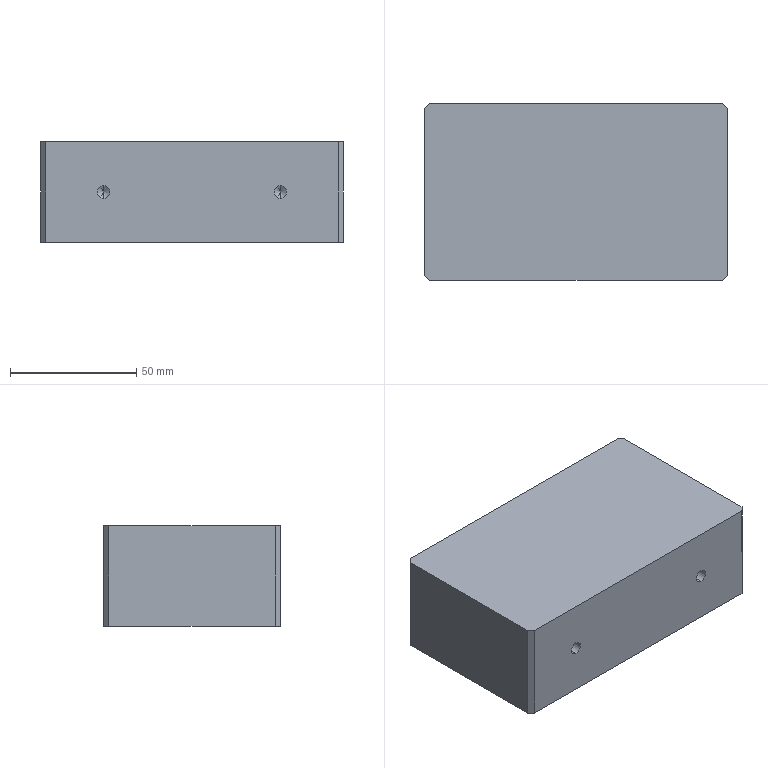Component | SolidWorks | ThirdGenerationFour-sidedLabelingFeedingSupportPlate-1 | 1 solid | 34 faces | box 120 x 70 x 40 mm | volume 334028 mm3 | cylinder 12 | cone 12 | plane 10 | commonest cylinder face diameters 4.2 x8 5 x4
build123d program:
from build123d import *

# Parameters (mm, degrees)
SKETCH1_W                  = 120
SKETCH1_H                  = 70
BOSS_EXTRUDE1_DEPTH        = 20
M5_TAPPED_HOLE1_AT_2_COUNT = 2
M5_TAPPED_HOLE1_AT_2_PITCH = 100
M6_TAPPED_HOLE1_AT_2_COUNT = 2
M6_TAPPED_HOLE1_AT_2_PITCH = 70
CHAMFER1_SIZE              = 2


with BuildPart() as part:
    # Sketch1 → Boss-Extrude1 (new, symmetric)
    with BuildSketch(Plane.XY):
        Rectangle(SKETCH1_W, SKETCH1_H)
    extrude(amount=BOSS_EXTRUDE1_DEPTH, both=True)

    # Sketch2 → M5 Tapped Hole1 (revolve, cut)
    with BuildSketch(Plane(origin=(-50, 35, -12), x_dir=(0, 0, 1), z_dir=(1, 0, 0))):
        Polygon((0, 0), (0, 19.662), (2.1, 18.4), (2.1, 0), align=None)
    m5_tapped_hole1 = revolve(axis=Axis((-50, 41.35, -12), (0, -1, 0)), mode=Mode.SUBTRACT)

    # M5 Tapped Hole1 at 2: M5 Tapped Hole1 ×2
    with Locations(*[(i * M5_TAPPED_HOLE1_AT_2_PITCH, 0, 0) for i in range(1, M5_TAPPED_HOLE1_AT_2_COUNT)]):
        add(m5_tapped_hole1, mode=Mode.SUBTRACT)

    # Sketch5 → M6 Tapped Hole1 (revolve, cut)
    with BuildSketch(Plane(origin=(-35, -35, 0), x_dir=(0, 0, -1), z_dir=(1, 0, 0))):
        Polygon((0, 0), (0, 16.502), (2.5, 15), (2.5, 0), align=None)
    m6_tapped_hole1 = revolve(axis=Axis((-35, -41.35, 0), (0, 1, 0)), mode=Mode.SUBTRACT)

    # M6 Tapped Hole1 at 2: M6 Tapped Hole1 ×2
    with Locations(*[(i * M6_TAPPED_HOLE1_AT_2_PITCH, 0, 0) for i in range(1, M6_TAPPED_HOLE1_AT_2_COUNT)]):
        add(m6_tapped_hole1, mode=Mode.SUBTRACT)

    # Chamfer1
    chamfer1_edges = [part.edges().sort_by_distance(p)[0] for p in [
        (60, -35, 0),
        (-60, -35, 0),
        (-60, 35, 0),
        (60, 35, 0),
    ]]
    chamfer(chamfer1_edges, length=CHAMFER1_SIZE)

    # Mirror1: M5 Tapped Hole1, M6 Tapped Hole1 across plane
    add(m5_tapped_hole1.mirror(Plane.XY), mode=Mode.SUBTRACT)
    add(m6_tapped_hole1.mirror(Plane.XY), mode=Mode.SUBTRACT)

    # Mirror1 copy 1 sketch → Mirror1 copy 1 (revolve, cut)
    with BuildSketch(Plane(origin=(50, 35, 12), x_dir=(0, 0, -1), z_dir=(1, 0, 0))):
        Polygon((0, 0), (0, -19.662), (2.1, -18.4), (2.1, 0), align=None)
    revolve(axis=Axis((50, 41.35, 12), (0, 1, 0)), mode=Mode.SUBTRACT)

    # Mirror1 copy 2 sketch → Mirror1 copy 2 (revolve, cut)
    with BuildSketch(Plane(origin=(35, -35, 0), x_dir=(0, 0, 1), z_dir=(1, 0, 0))):
        Polygon((0, 0), (0, -16.502), (2.5, -15), (2.5, 0), align=None)
    revolve(axis=Axis((35, -41.35, 0), (0, -1, 0)), mode=Mode.SUBTRACT)


solid = part.part

# Placed as in the assembly
solid = solid.moved(Location((-20.027, -1.137, 0), (0, 0, 0)))
STEP:
#1=CARTESIAN_POINT('',(-2.757,0.6088,0.3898));
#2=VERTEX_POINT('',#1);
#3=CARTESIAN_POINT('',(-2.757,0.6088,0.5551));
#4=VERTEX_POINT('',#3);
#5=CARTESIAN_POINT('',(-2.757,0.6088,0.4724));
#6=DIRECTION('',(0.,1.,0.));
#7=DIRECTION('',(0.,0.,1.));
#8=AXIS2_PLACEMENT_3D('',#5,#6,#7);
#9=CIRCLE('',#8,0.08268);
#10=EDGE_CURVE('',#2,#4,#9,.T.);
#11=ORIENTED_EDGE('',*,*,#10,.F.);
#12=CARTESIAN_POINT('',(-2.757,1.333,0.3898));
#13=VERTEX_POINT('',#12);
#14=CARTESIAN_POINT('',(-2.757,1.333,0.3898));
#15=DIRECTION('',(0.,1.,0.));
#16=VECTOR('',#15,39.37);
#17=LINE('',#14,#16);
#18=EDGE_CURVE('',#2,#13,#17,.T.);
#19=ORIENTED_EDGE('',*,*,#18,.T.);
#20=CARTESIAN_POINT('',(-2.757,1.333,0.5551));
#21=VERTEX_POINT('',#20);
#22=CARTESIAN_POINT('',(-2.757,1.333,0.4724));
#23=DIRECTION('',(0.,1.,0.));
#24=DIRECTION('',(0.,0.,1.));
#25=AXIS2_PLACEMENT_3D('',#22,#23,#24);
#26=CIRCLE('',#25,0.08268);
#27=EDGE_CURVE('',#13,#21,#26,.T.);
#28=ORIENTED_EDGE('',*,*,#27,.T.);
#29=CARTESIAN_POINT('',(-2.757,1.333,0.5551));
#30=DIRECTION('',(0.,1.,0.));
#31=VECTOR('',#30,39.37);
#32=LINE('',#29,#31);
#33=EDGE_CURVE('',#4,#21,#32,.T.);
#34=ORIENTED_EDGE('',*,*,#33,.F.);
#35=EDGE_LOOP('',(#11,#19,#28,#34));
#36=FACE_OUTER_BOUND('',#35,.T.);
#37=CARTESIAN_POINT('',(-2.757,1.333,0.4724));
#38=DIRECTION('',(0.,1.,0.));
#39=DIRECTION('',(0.,0.,1.));
#40=AXIS2_PLACEMENT_3D('',#37,#38,#39);
#41=CYLINDRICAL_SURFACE('',#40,0.08268);
#42=ADVANCED_FACE('',(#36),#41,.F.);
#43=CARTESIAN_POINT('',(-2.757,0.5591,0.4724));
#44=VERTEX_POINT('',#43);
#45=CARTESIAN_POINT('',(-2.757,0.6088,0.5551));
#46=DIRECTION('',(0.,0.515,0.8572));
#47=VECTOR('',#46,39.37);
#48=LINE('',#45,#47);
#49=EDGE_CURVE('',#44,#4,#48,.T.);
#50=ORIENTED_EDGE('',*,*,#49,.F.);
#51=CARTESIAN_POINT('',(-2.757,0.6088,0.3898));
#52=DIRECTION('',(0.,0.515,-0.8572));
#53=VECTOR('',#52,39.37);
#54=LINE('',#51,#53);
#55=EDGE_CURVE('',#44,#2,#54,.T.);
#56=ORIENTED_EDGE('',*,*,#55,.T.);
#57=ORIENTED_EDGE('',*,*,#10,.T.);
#58=EDGE_LOOP('',(#50,#56,#57));
#59=FACE_OUTER_BOUND('',#58,.T.);
#60=CARTESIAN_POINT('',(-2.757,0.6088,0.4724));
#61=DIRECTION('',(0.,1.,0.));
#62=DIRECTION('',(0.,0.,1.));
#63=AXIS2_PLACEMENT_3D('',#60,#61,#62);
#64=CONICAL_SURFACE('',#63,0.08268,1.03);
#65=ADVANCED_FACE('',(#59),#64,.F.);
#66=CARTESIAN_POINT('',(1.18,0.6088,0.3898));
#67=VERTEX_POINT('',#66);
#68=CARTESIAN_POINT('',(1.18,0.6088,0.5551));
#69=VERTEX_POINT('',#68);
#70=CARTESIAN_POINT('',(1.18,0.6088,0.4724));
#71=DIRECTION('',(0.,1.,0.));
#72=DIRECTION('',(0.,0.,1.));
#73=AXIS2_PLACEMENT_3D('',#70,#71,#72);
#74=CIRCLE('',#73,0.08268);
#75=EDGE_CURVE('',#67,#69,#74,.T.);
#76=ORIENTED_EDGE('',*,*,#75,.F.);
#77=CARTESIAN_POINT('',(1.18,1.333,0.3898));
#78=VERTEX_POINT('',#77);
#79=CARTESIAN_POINT('',(1.18,1.333,0.3898));
#80=DIRECTION('',(0.,1.,0.));
#81=VECTOR('',#80,39.37);
#82=LINE('',#79,#81);
#83=EDGE_CURVE('',#67,#78,#82,.T.);
#84=ORIENTED_EDGE('',*,*,#83,.T.);
#85=CARTESIAN_POINT('',(1.18,1.333,0.5551));
#86=VERTEX_POINT('',#85);
#87=CARTESIAN_POINT('',(1.18,1.333,0.4724));
#88=DIRECTION('',(0.,1.,0.));
#89=DIRECTION('',(0.,0.,1.));
#90=AXIS2_PLACEMENT_3D('',#87,#88,#89);
#91=CIRCLE('',#90,0.08268);
#92=EDGE_CURVE('',#78,#86,#91,.T.);
#93=ORIENTED_EDGE('',*,*,#92,.T.);
#94=CARTESIAN_POINT('',(1.18,1.333,0.5551));
#95=DIRECTION('',(0.,1.,0.));
#96=VECTOR('',#95,39.37);
#97=LINE('',#94,#96);
#98=EDGE_CURVE('',#69,#86,#97,.T.);
#99=ORIENTED_EDGE('',*,*,#98,.F.);
#100=EDGE_LOOP('',(#76,#84,#93,#99));
#101=FACE_OUTER_BOUND('',#100,.T.);
#102=CARTESIAN_POINT('',(1.18,1.333,0.4724));
#103=DIRECTION('',(0.,1.,0.));
#104=DIRECTION('',(0.,0.,1.));
#105=AXIS2_PLACEMENT_3D('',#102,#103,#104);
#106=CYLINDRICAL_SURFACE('',#105,0.08268);
#107=ADVANCED_FACE('',(#101),#106,.F.);
#108=CARTESIAN_POINT('',(1.18,0.5591,0.4724));
#109=VERTEX_POINT('',#108);
#110=CARTESIAN_POINT('',(1.18,0.6088,0.5551));
#111=DIRECTION('',(0.,0.515,0.8572));
#112=VECTOR('',#111,39.37);
#113=LINE('',#110,#112);
#114=EDGE_CURVE('',#109,#69,#113,.T.);
#115=ORIENTED_EDGE('',*,*,#114,.F.);
#116=CARTESIAN_POINT('',(1.18,0.6088,0.3898));
#117=DIRECTION('',(0.,0.515,-0.8572));
#118=VECTOR('',#117,39.37);
#119=LINE('',#116,#118);
#120=EDGE_CURVE('',#109,#67,#119,.T.);
#121=ORIENTED_EDGE('',*,*,#120,.T.);
#122=ORIENTED_EDGE('',*,*,#75,.T.);
#123=EDGE_LOOP('',(#115,#121,#122));
#124=FACE_OUTER_BOUND('',#123,.T.);
#125=CARTESIAN_POINT('',(1.18,0.6088,0.4724));
#126=DIRECTION('',(0.,1.,0.));
#127=DIRECTION('',(0.,0.,1.));
#128=AXIS2_PLACEMENT_3D('',#125,#126,#127);
#129=CONICAL_SURFACE('',#128,0.08268,1.03);
#130=ADVANCED_FACE('',(#124),#129,.F.);
#131=CARTESIAN_POINT('',(-2.166,-0.8322,0.09843));
#132=VERTEX_POINT('',#131);
#133=CARTESIAN_POINT('',(-2.166,-0.8322,-0.09843));
#134=VERTEX_POINT('',#133);
#135=CARTESIAN_POINT('',(-2.166,-0.8322,0.));
#136=DIRECTION('',(0.,-1.,0.));
#137=DIRECTION('',(0.,0.,-1.));
#138=AXIS2_PLACEMENT_3D('',#135,#136,#137);
#139=CIRCLE('',#138,0.09843);
#140=EDGE_CURVE('',#132,#134,#139,.T.);
#141=ORIENTED_EDGE('',*,*,#140,.F.);
#142=CARTESIAN_POINT('',(-2.166,-1.423,0.09843));
#143=VERTEX_POINT('',#142);
#144=CARTESIAN_POINT('',(-2.166,-1.423,0.09843));
#145=DIRECTION('',(0.,-1.,0.));
#146=VECTOR('',#145,39.37);
#147=LINE('',#144,#146);
#148=EDGE_CURVE('',#132,#143,#147,.T.);
#149=ORIENTED_EDGE('',*,*,#148,.T.);
#150=CARTESIAN_POINT('',(-2.166,-1.423,-0.09843));
#151=VERTEX_POINT('',#150);
#152=CARTESIAN_POINT('',(-2.166,-1.423,0.));
#153=DIRECTION('',(0.,-1.,0.));
#154=DIRECTION('',(0.,0.,-1.));
#155=AXIS2_PLACEMENT_3D('',#152,#153,#154);
#156=CIRCLE('',#155,0.09843);
#157=EDGE_CURVE('',#143,#151,#156,.T.);
#158=ORIENTED_EDGE('',*,*,#157,.T.);
#159=CARTESIAN_POINT('',(-2.166,-1.423,-0.09843));
#160=DIRECTION('',(0.,-1.,0.));
#161=VECTOR('',#160,39.37);
#162=LINE('',#159,#161);
#163=EDGE_CURVE('',#134,#151,#162,.T.);
#164=ORIENTED_EDGE('',*,*,#163,.F.);
#165=EDGE_LOOP('',(#141,#149,#158,#164));
#166=FACE_OUTER_BOUND('',#165,.T.);
#167=CARTESIAN_POINT('',(-2.166,-1.423,0.));
#168=DIRECTION('',(0.,-1.,0.));
#169=DIRECTION('',(0.,0.,-1.));
#170=AXIS2_PLACEMENT_3D('',#167,#168,#169);
#171=CYLINDRICAL_SURFACE('',#170,0.09843);
#172=ADVANCED_FACE('',(#166),#171,.F.);
#173=CARTESIAN_POINT('',(-2.166,-0.773,0.));
#174=VERTEX_POINT('',#173);
#175=CARTESIAN_POINT('',(-2.166,-0.8322,-0.09843));
#176=DIRECTION('',(0.,-0.515,-0.8572));
#177=VECTOR('',#176,39.37);
#178=LINE('',#175,#177);
#179=EDGE_CURVE('',#174,#134,#178,.T.);
#180=ORIENTED_EDGE('',*,*,#179,.F.);
#181=CARTESIAN_POINT('',(-2.166,-0.8322,0.09843));
#182=DIRECTION('',(0.,-0.515,0.8572));
#183=VECTOR('',#182,39.37);
#184=LINE('',#181,#183);
#185=EDGE_CURVE('',#174,#132,#184,.T.);
#186=ORIENTED_EDGE('',*,*,#185,.T.);
#187=ORIENTED_EDGE('',*,*,#140,.T.);
#188=EDGE_LOOP('',(#180,#186,#187));
#189=FACE_OUTER_BOUND('',#188,.T.);
#190=CARTESIAN_POINT('',(-2.166,-0.8322,0.));
#191=DIRECTION('',(0.,-1.,0.));
#192=DIRECTION('',(0.,0.,-1.));
#193=AXIS2_PLACEMENT_3D('',#190,#191,#192);
#194=CONICAL_SURFACE('',#193,0.09843,1.03);
#195=ADVANCED_FACE('',(#189),#194,.F.);
#196=CARTESIAN_POINT('',(0.5895,-0.8322,0.09843));
#197=VERTEX_POINT('',#196);
#198=CARTESIAN_POINT('',(0.5895,-0.8322,-0.09843));
#199=VERTEX_POINT('',#198);
#200=CARTESIAN_POINT('',(0.5895,-0.8322,0.));
#201=DIRECTION('',(0.,-1.,0.));
#202=DIRECTION('',(0.,0.,-1.));
#203=AXIS2_PLACEMENT_3D('',#200,#201,#202);
#204=CIRCLE('',#203,0.09843);
#205=EDGE_CURVE('',#197,#199,#204,.T.);
#206=ORIENTED_EDGE('',*,*,#205,.F.);
#207=CARTESIAN_POINT('',(0.5895,-1.423,0.09843));
#208=VERTEX_POINT('',#207);
#209=CARTESIAN_POINT('',(0.5895,-1.423,0.09843));
#210=DIRECTION('',(0.,-1.,0.));
#211=VECTOR('',#210,39.37);
#212=LINE('',#209,#211);
#213=EDGE_CURVE('',#197,#208,#212,.T.);
#214=ORIENTED_EDGE('',*,*,#213,.T.);
#215=CARTESIAN_POINT('',(0.5895,-1.423,-0.09843));
#216=VERTEX_POINT('',#215);
#217=CARTESIAN_POINT('',(0.5895,-1.423,0.));
#218=DIRECTION('',(0.,-1.,0.));
#219=DIRECTION('',(0.,0.,-1.));
#220=AXIS2_PLACEMENT_3D('',#217,#218,#219);
#221=CIRCLE('',#220,0.09843);
#222=EDGE_CURVE('',#208,#216,#221,.T.);
#223=ORIENTED_EDGE('',*,*,#222,.T.);
#224=CARTESIAN_POINT('',(0.5895,-1.423,-0.09843));
#225=DIRECTION('',(0.,-1.,0.));
#226=VECTOR('',#225,39.37);
#227=LINE('',#224,#226);
#228=EDGE_CURVE('',#199,#216,#227,.T.);
#229=ORIENTED_EDGE('',*,*,#228,.F.);
#230=EDGE_LOOP('',(#206,#214,#223,#229));
#231=FACE_OUTER_BOUND('',#230,.T.);
#232=CARTESIAN_POINT('',(0.5895,-1.423,0.));
#233=DIRECTION('',(0.,-1.,0.));
#234=DIRECTION('',(0.,0.,-1.));
#235=AXIS2_PLACEMENT_3D('',#232,#233,#234);
#236=CYLINDRICAL_SURFACE('',#235,0.09843);
#237=ADVANCED_FACE('',(#231),#236,.F.);
#238=CARTESIAN_POINT('',(0.5895,-0.773,0.));
#239=VERTEX_POINT('',#238);
#240=CARTESIAN_POINT('',(0.5895,-0.8322,-0.09843));
#241=DIRECTION('',(0.,-0.515,-0.8572));
#242=VECTOR('',#241,39.37);
#243=LINE('',#240,#242);
#244=EDGE_CURVE('',#239,#199,#243,.T.);
#245=ORIENTED_EDGE('',*,*,#244,.F.);
#246=CARTESIAN_POINT('',(0.5895,-0.8322,0.09843));
#247=DIRECTION('',(0.,-0.515,0.8572));
#248=VECTOR('',#247,39.37);
#249=LINE('',#246,#248);
#250=EDGE_CURVE('',#239,#197,#249,.T.);
#251=ORIENTED_EDGE('',*,*,#250,.T.);
#252=ORIENTED_EDGE('',*,*,#205,.T.);
#253=EDGE_LOOP('',(#245,#251,#252));
#254=FACE_OUTER_BOUND('',#253,.T.);
#255=CARTESIAN_POINT('',(0.5895,-0.8322,0.));
#256=DIRECTION('',(0.,-1.,0.));
#257=DIRECTION('',(0.,0.,-1.));
#258=AXIS2_PLACEMENT_3D('',#255,#256,#257);
#259=CONICAL_SURFACE('',#258,0.09843,1.03);
#260=ADVANCED_FACE('',(#254),#259,.F.);
#261=CARTESIAN_POINT('',(-2.757,0.6088,-0.5551));
#262=VERTEX_POINT('',#261);
#263=CARTESIAN_POINT('',(-2.757,0.6088,-0.3898));
#264=VERTEX_POINT('',#263);
#265=CARTESIAN_POINT('',(-2.757,0.6088,-0.4724));
#266=DIRECTION('',(0.,1.,0.));
#267=DIRECTION('',(0.,0.,1.));
#268=AXIS2_PLACEMENT_3D('',#265,#266,#267);
#269=CIRCLE('',#268,0.08268);
#270=EDGE_CURVE('',#262,#264,#269,.T.);
#271=ORIENTED_EDGE('',*,*,#270,.F.);
#272=CARTESIAN_POINT('',(-2.757,1.333,-0.5551));
#273=VERTEX_POINT('',#272);
#274=CARTESIAN_POINT('',(-2.757,1.333,-0.5551));
#275=DIRECTION('',(0.,1.,0.));
#276=VECTOR('',#275,39.37);
#277=LINE('',#274,#276);
#278=EDGE_CURVE('',#262,#273,#277,.T.);
#279=ORIENTED_EDGE('',*,*,#278,.T.);
#280=CARTESIAN_POINT('',(-2.757,1.333,-0.3898));
#281=VERTEX_POINT('',#280);
#282=CARTESIAN_POINT('',(-2.757,1.333,-0.4724));
#283=DIRECTION('',(0.,1.,0.));
#284=DIRECTION('',(0.,0.,1.));
#285=AXIS2_PLACEMENT_3D('',#282,#283,#284);
#286=CIRCLE('',#285,0.08268);
#287=EDGE_CURVE('',#273,#281,#286,.T.);
#288=ORIENTED_EDGE('',*,*,#287,.T.);
#289=CARTESIAN_POINT('',(-2.757,1.333,-0.3898));
#290=DIRECTION('',(0.,1.,0.));
#291=VECTOR('',#290,39.37);
#292=LINE('',#289,#291);
#293=EDGE_CURVE('',#264,#281,#292,.T.);
#294=ORIENTED_EDGE('',*,*,#293,.F.);
#295=EDGE_LOOP('',(#271,#279,#288,#294));
#296=FACE_OUTER_BOUND('',#295,.T.);
#297=CARTESIAN_POINT('',(-2.757,1.333,-0.4724));
#298=DIRECTION('',(0.,1.,0.));
#299=DIRECTION('',(0.,0.,1.));
#300=AXIS2_PLACEMENT_3D('',#297,#298,#299);
#301=CYLINDRICAL_SURFACE('',#300,0.08268);
#302=ADVANCED_FACE('',(#296),#301,.F.);
#303=CARTESIAN_POINT('',(-2.757,0.5591,-0.4724));
#304=VERTEX_POINT('',#303);
#305=CARTESIAN_POINT('',(-2.757,0.6088,-0.3898));
#306=DIRECTION('',(0.,0.515,0.8572));
#307=VECTOR('',#306,39.37);
#308=LINE('',#305,#307);
#309=EDGE_CURVE('',#304,#264,#308,.T.);
#310=ORIENTED_EDGE('',*,*,#309,.F.);
#311=CARTESIAN_POINT('',(-2.757,0.6088,-0.5551));
#312=DIRECTION('',(0.,0.515,-0.8572));
#313=VECTOR('',#312,39.37);
#314=LINE('',#311,#313);
#315=EDGE_CURVE('',#304,#262,#314,.T.);
#316=ORIENTED_EDGE('',*,*,#315,.T.);
#317=ORIENTED_EDGE('',*,*,#270,.T.);
#318=EDGE_LOOP('',(#310,#316,#317));
#319=FACE_OUTER_BOUND('',#318,.T.);
#320=CARTESIAN_POINT('',(-2.757,0.6088,-0.4724));
#321=DIRECTION('',(0.,1.,0.));
#322=DIRECTION('',(0.,0.,1.));
#323=AXIS2_PLACEMENT_3D('',#320,#321,#322);
#324=CONICAL_SURFACE('',#323,0.08268,1.03);
#325=ADVANCED_FACE('',(#319),#324,.F.);
#326=CARTESIAN_POINT('',(1.18,0.6088,-0.5551));
#327=VERTEX_POINT('',#326);
#328=CARTESIAN_POINT('',(1.18,0.6088,-0.3898));
#329=VERTEX_POINT('',#328);
#330=CARTESIAN_POINT('',(1.18,0.6088,-0.4724));
#331=DIRECTION('',(0.,1.,0.));
#332=DIRECTION('',(0.,0.,1.));
#333=AXIS2_PLACEMENT_3D('',#330,#331,#332);
#334=CIRCLE('',#333,0.08268);
#335=EDGE_CURVE('',#327,#329,#334,.T.);
#336=ORIENTED_EDGE('',*,*,#335,.F.);
#337=CARTESIAN_POINT('',(1.18,1.333,-0.5551));
#338=VERTEX_POINT('',#337);
#339=CARTESIAN_POINT('',(1.18,1.333,-0.5551));
#340=DIRECTION('',(0.,1.,0.));
#341=VECTOR('',#340,39.37);
#342=LINE('',#339,#341);
#343=EDGE_CURVE('',#327,#338,#342,.T.);
#344=ORIENTED_EDGE('',*,*,#343,.T.);
#345=CARTESIAN_POINT('',(1.18,1.333,-0.3898));
#346=VERTEX_POINT('',#345);
#347=CARTESIAN_POINT('',(1.18,1.333,-0.4724));
#348=DIRECTION('',(0.,1.,0.));
#349=DIRECTION('',(0.,0.,1.));
#350=AXIS2_PLACEMENT_3D('',#347,#348,#349);
#351=CIRCLE('',#350,0.08268);
#352=EDGE_CURVE('',#338,#346,#351,.T.);
#353=ORIENTED_EDGE('',*,*,#352,.T.);
#354=CARTESIAN_POINT('',(1.18,1.333,-0.3898));
#355=DIRECTION('',(0.,1.,0.));
#356=VECTOR('',#355,39.37);
#357=LINE('',#354,#356);
#358=EDGE_CURVE('',#329,#346,#357,.T.);
#359=ORIENTED_EDGE('',*,*,#358,.F.);
#360=EDGE_LOOP('',(#336,#344,#353,#359));
#361=FACE_OUTER_BOUND('',#360,.T.);
#362=CARTESIAN_POINT('',(1.18,1.333,-0.4724));
#363=DIRECTION('',(0.,1.,0.));
#364=DIRECTION('',(0.,0.,1.));
#365=AXIS2_PLACEMENT_3D('',#362,#363,#364);
#366=CYLINDRICAL_SURFACE('',#365,0.08268);
#367=ADVANCED_FACE('',(#361),#366,.F.);
#368=CARTESIAN_POINT('',(1.18,0.5591,-0.4724));
#369=VERTEX_POINT('',#368);
#370=CARTESIAN_POINT('',(1.18,0.6088,-0.3898));
#371=DIRECTION('',(0.,0.515,0.8572));
#372=VECTOR('',#371,39.37);
#373=LINE('',#370,#372);
#374=EDGE_CURVE('',#369,#329,#373,.T.);
#375=ORIENTED_EDGE('',*,*,#374,.F.);
#376=CARTESIAN_POINT('',(1.18,0.6088,-0.5551));
#377=DIRECTION('',(0.,0.515,-0.8572));
#378=VECTOR('',#377,39.37);
#379=LINE('',#376,#378);
#380=EDGE_CURVE('',#369,#327,#379,.T.);
#381=ORIENTED_EDGE('',*,*,#380,.T.);
#382=ORIENTED_EDGE('',*,*,#335,.T.);
#383=EDGE_LOOP('',(#375,#381,#382));
#384=FACE_OUTER_BOUND('',#383,.T.);
#385=CARTESIAN_POINT('',(1.18,0.6088,-0.4724));
#386=DIRECTION('',(0.,1.,0.));
#387=DIRECTION('',(0.,0.,1.));
#388=AXIS2_PLACEMENT_3D('',#385,#386,#387);
#389=CONICAL_SURFACE('',#388,0.08268,1.03);
#390=ADVANCED_FACE('',(#384),#389,.F.);
#391=CARTESIAN_POINT('',(1.574,-1.344,-0.7874));
#392=VERTEX_POINT('',#391);
#393=CARTESIAN_POINT('',(1.574,1.254,-0.7874));
#394=VERTEX_POINT('',#393);
#395=CARTESIAN_POINT('',(1.574,-1.423,-0.7874));
#396=DIRECTION('',(0.,1.,0.));
#397=VECTOR('',#396,39.37);
#398=LINE('',#395,#397);
#399=EDGE_CURVE('',#392,#394,#398,.T.);
#400=ORIENTED_EDGE('',*,*,#399,.T.);
#401=CARTESIAN_POINT('',(1.574,1.254,0.7874));
#402=VERTEX_POINT('',#401);
#403=CARTESIAN_POINT('',(1.574,1.254,0.7874));
#404=DIRECTION('',(0.,0.,1.));
#405=VECTOR('',#404,39.37);
#406=LINE('',#403,#405);
#407=EDGE_CURVE('',#394,#402,#406,.T.);
#408=ORIENTED_EDGE('',*,*,#407,.T.);
#409=CARTESIAN_POINT('',(1.574,-1.344,0.7874));
#410=VERTEX_POINT('',#409);
#411=CARTESIAN_POINT('',(1.574,-1.423,0.7874));
#412=DIRECTION('',(0.,1.,0.));
#413=VECTOR('',#412,39.37);
#414=LINE('',#411,#413);
#415=EDGE_CURVE('',#410,#402,#414,.T.);
#416=ORIENTED_EDGE('',*,*,#415,.F.);
#417=CARTESIAN_POINT('',(1.574,-1.344,0.7874));
#418=DIRECTION('',(0.,0.,-1.));
#419=VECTOR('',#418,39.37);
#420=LINE('',#417,#419);
#421=EDGE_CURVE('',#410,#392,#420,.T.);
#422=ORIENTED_EDGE('',*,*,#421,.T.);
#423=EDGE_LOOP('',(#400,#408,#416,#422));
#424=FACE_OUTER_BOUND('',#423,.T.);
#425=CARTESIAN_POINT('',(1.574,-1.423,0.7874));
#426=DIRECTION('',(-1.,0.,0.));
#427=DIRECTION('',(0.,0.,1.));
#428=AXIS2_PLACEMENT_3D('',#425,#426,#427);
#429=PLANE('',#428);
#430=ADVANCED_FACE('',(#424),#429,.F.);
#431=CARTESIAN_POINT('',(-2.757,1.333,0.4724));
#432=DIRECTION('',(0.,1.,0.));
#433=DIRECTION('',(0.,0.,1.));
#434=AXIS2_PLACEMENT_3D('',#431,#432,#433);
#435=CIRCLE('',#434,0.08268);
#436=EDGE_CURVE('',#21,#13,#435,.T.);
#437=ORIENTED_EDGE('',*,*,#436,.F.);
#438=ORIENTED_EDGE('',*,*,#27,.F.);
#439=EDGE_LOOP('',(#437,#438));
#440=FACE_BOUND('',#439,.T.);
#441=CARTESIAN_POINT('',(1.18,1.333,0.4724));
#442=DIRECTION('',(0.,1.,0.));
#443=DIRECTION('',(0.,0.,1.));
#444=AXIS2_PLACEMENT_3D('',#441,#442,#443);
#445=CIRCLE('',#444,0.08268);
#446=EDGE_CURVE('',#86,#78,#445,.T.);
#447=ORIENTED_EDGE('',*,*,#446,.F.);
#448=ORIENTED_EDGE('',*,*,#92,.F.);
#449=EDGE_LOOP('',(#447,#448));
#450=FACE_BOUND('',#449,.T.);
#451=CARTESIAN_POINT('',(-2.757,1.333,-0.4724));
#452=DIRECTION('',(0.,1.,0.));
#453=DIRECTION('',(0.,0.,1.));
#454=AXIS2_PLACEMENT_3D('',#451,#452,#453);
#455=CIRCLE('',#454,0.08268);
#456=EDGE_CURVE('',#281,#273,#455,.T.);
#457=ORIENTED_EDGE('',*,*,#456,.F.);
#458=ORIENTED_EDGE('',*,*,#287,.F.);
#459=EDGE_LOOP('',(#457,#458));
#460=FACE_BOUND('',#459,.T.);
#461=CARTESIAN_POINT('',(1.18,1.333,-0.4724));
#462=DIRECTION('',(0.,1.,0.));
#463=DIRECTION('',(0.,0.,1.));
#464=AXIS2_PLACEMENT_3D('',#461,#462,#463);
#465=CIRCLE('',#464,0.08268);
#466=EDGE_CURVE('',#346,#338,#465,.T.);
#467=ORIENTED_EDGE('',*,*,#466,.F.);
#468=ORIENTED_EDGE('',*,*,#352,.F.);
#469=EDGE_LOOP('',(#467,#468));
#470=FACE_BOUND('',#469,.T.);
#471=CARTESIAN_POINT('',(1.495,1.333,0.7874));
#472=VERTEX_POINT('',#471);
#473=CARTESIAN_POINT('',(-3.072,1.333,0.7874));
#474=VERTEX_POINT('',#473);
#475=CARTESIAN_POINT('',(-3.151,1.333,0.7874));
#476=DIRECTION('',(-1.,0.,0.));
#477=VECTOR('',#476,39.37);
#478=LINE('',#475,#477);
#479=EDGE_CURVE('',#472,#474,#478,.T.);
#480=ORIENTED_EDGE('',*,*,#479,.F.);
#481=CARTESIAN_POINT('',(1.495,1.333,-0.7874));
#482=VERTEX_POINT('',#481);
#483=CARTESIAN_POINT('',(1.495,1.333,0.7874));
#484=DIRECTION('',(0.,0.,-1.));
#485=VECTOR('',#484,39.37);
#486=LINE('',#483,#485);
#487=EDGE_CURVE('',#472,#482,#486,.T.);
#488=ORIENTED_EDGE('',*,*,#487,.T.);
#489=CARTESIAN_POINT('',(-3.072,1.333,-0.7874));
#490=VERTEX_POINT('',#489);
#491=CARTESIAN_POINT('',(-3.151,1.333,-0.7874));
#492=DIRECTION('',(-1.,0.,0.));
#493=VECTOR('',#492,39.37);
#494=LINE('',#491,#493);
#495=EDGE_CURVE('',#482,#490,#494,.T.);
#496=ORIENTED_EDGE('',*,*,#495,.T.);
#497=CARTESIAN_POINT('',(-3.072,1.333,0.7874));
#498=DIRECTION('',(0.,0.,1.));
#499=VECTOR('',#498,39.37);
#500=LINE('',#497,#499);
#501=EDGE_CURVE('',#490,#474,#500,.T.);
#502=ORIENTED_EDGE('',*,*,#501,.T.);
#503=EDGE_LOOP('',(#480,#488,#496,#502));
#504=FACE_OUTER_BOUND('',#503,.T.);
#505=CARTESIAN_POINT('',(-3.151,1.333,0.7874));
#506=DIRECTION('',(0.,-1.,0.));
#507=DIRECTION('',(0.,0.,-1.));
#508=AXIS2_PLACEMENT_3D('',#505,#506,#507);
#509=PLANE('',#508);
#510=ADVANCED_FACE('',(#440,#450,#460,#470,#504),#509,.F.);
#511=CARTESIAN_POINT('',(-3.151,1.254,-0.7874));
#512=VERTEX_POINT('',#511);
#513=CARTESIAN_POINT('',(-3.151,-1.344,-0.7874));
#514=VERTEX_POINT('',#513);
#515=CARTESIAN_POINT('',(-3.151,-1.423,-0.7874));
#516=DIRECTION('',(0.,-1.,0.));
#517=VECTOR('',#516,39.37);
#518=LINE('',#515,#517);
#519=EDGE_CURVE('',#512,#514,#518,.T.);
#520=ORIENTED_EDGE('',*,*,#519,.T.);
#521=CARTESIAN_POINT('',(-3.151,-1.344,0.7874));
#522=VERTEX_POINT('',#521);
#523=CARTESIAN_POINT('',(-3.151,-1.344,0.7874));
#524=DIRECTION('',(0.,0.,1.));
#525=VECTOR('',#524,39.37);
#526=LINE('',#523,#525);
#527=EDGE_CURVE('',#514,#522,#526,.T.);
#528=ORIENTED_EDGE('',*,*,#527,.T.);
#529=CARTESIAN_POINT('',(-3.151,1.254,0.7874));
#530=VERTEX_POINT('',#529);
#531=CARTESIAN_POINT('',(-3.151,-1.423,0.7874));
#532=DIRECTION('',(0.,-1.,0.));
#533=VECTOR('',#532,39.37);
#534=LINE('',#531,#533);
#535=EDGE_CURVE('',#530,#522,#534,.T.);
#536=ORIENTED_EDGE('',*,*,#535,.F.);
#537=CARTESIAN_POINT('',(-3.151,1.254,0.7874));
#538=DIRECTION('',(0.,0.,-1.));
#539=VECTOR('',#538,39.37);
#540=LINE('',#537,#539);
#541=EDGE_CURVE('',#530,#512,#540,.T.);
#542=ORIENTED_EDGE('',*,*,#541,.T.);
#543=EDGE_LOOP('',(#520,#528,#536,#542));
#544=FACE_OUTER_BOUND('',#543,.T.);
#545=CARTESIAN_POINT('',(-3.151,-1.423,0.7874));
#546=DIRECTION('',(1.,0.,0.));
#547=DIRECTION('',(0.,0.,-1.));
#548=AXIS2_PLACEMENT_3D('',#545,#546,#547);
#549=PLANE('',#548);
#550=ADVANCED_FACE('',(#544),#549,.F.);
#551=CARTESIAN_POINT('',(-2.166,-1.423,0.));
#552=DIRECTION('',(0.,-1.,0.));
#553=DIRECTION('',(0.,0.,-1.));
#554=AXIS2_PLACEMENT_3D('',#551,#552,#553);
#555=CIRCLE('',#554,0.09843);
#556=EDGE_CURVE('',#151,#143,#555,.T.);
#557=ORIENTED_EDGE('',*,*,#556,.F.);
#558=ORIENTED_EDGE('',*,*,#157,.F.);
#559=EDGE_LOOP('',(#557,#558));
#560=FACE_BOUND('',#559,.T.);
#561=CARTESIAN_POINT('',(0.5895,-1.423,0.));
#562=DIRECTION('',(0.,-1.,0.));
#563=DIRECTION('',(0.,0.,-1.));
#564=AXIS2_PLACEMENT_3D('',#561,#562,#563);
#565=CIRCLE('',#564,0.09843);
#566=EDGE_CURVE('',#216,#208,#565,.T.);
#567=ORIENTED_EDGE('',*,*,#566,.F.);
#568=ORIENTED_EDGE('',*,*,#222,.F.);
#569=EDGE_LOOP('',(#567,#568));
#570=FACE_BOUND('',#569,.T.);
#571=CARTESIAN_POINT('',(-3.072,-1.423,-0.7874));
#572=VERTEX_POINT('',#571);
#573=CARTESIAN_POINT('',(1.495,-1.423,-0.7874));
#574=VERTEX_POINT('',#573);
#575=CARTESIAN_POINT('',(-3.151,-1.423,-0.7874));
#576=DIRECTION('',(1.,0.,0.));
#577=VECTOR('',#576,39.37);
#578=LINE('',#575,#577);
#579=EDGE_CURVE('',#572,#574,#578,.T.);
#580=ORIENTED_EDGE('',*,*,#579,.T.);
#581=CARTESIAN_POINT('',(1.495,-1.423,0.7874));
#582=VERTEX_POINT('',#581);
#583=CARTESIAN_POINT('',(1.495,-1.423,0.7874));
#584=DIRECTION('',(0.,0.,1.));
#585=VECTOR('',#584,39.37);
#586=LINE('',#583,#585);
#587=EDGE_CURVE('',#574,#582,#586,.T.);
#588=ORIENTED_EDGE('',*,*,#587,.T.);
#589=CARTESIAN_POINT('',(-3.072,-1.423,0.7874));
#590=VERTEX_POINT('',#589);
#591=CARTESIAN_POINT('',(-3.151,-1.423,0.7874));
#592=DIRECTION('',(1.,0.,0.));
#593=VECTOR('',#592,39.37);
#594=LINE('',#591,#593);
#595=EDGE_CURVE('',#590,#582,#594,.T.);
#596=ORIENTED_EDGE('',*,*,#595,.F.);
#597=CARTESIAN_POINT('',(-3.072,-1.423,0.7874));
#598=DIRECTION('',(0.,0.,-1.));
#599=VECTOR('',#598,39.37);
#600=LINE('',#597,#599);
#601=EDGE_CURVE('',#590,#572,#600,.T.);
#602=ORIENTED_EDGE('',*,*,#601,.T.);
#603=EDGE_LOOP('',(#580,#588,#596,#602));
#604=FACE_OUTER_BOUND('',#603,.T.);
#605=CARTESIAN_POINT('',(-3.151,-1.423,0.7874));
#606=DIRECTION('',(0.,1.,0.));
#607=DIRECTION('',(0.,0.,1.));
#608=AXIS2_PLACEMENT_3D('',#605,#606,#607);
#609=PLANE('',#608);
#610=ADVANCED_FACE('',(#560,#570,#604),#609,.F.);
#611=ORIENTED_EDGE('',*,*,#415,.T.);
#612=CARTESIAN_POINT('',(1.495,1.333,0.7874));
#613=DIRECTION('',(-0.7071,0.7071,0.));
#614=VECTOR('',#613,39.37);
#615=LINE('',#612,#614);
#616=EDGE_CURVE('',#402,#472,#615,.T.);
#617=ORIENTED_EDGE('',*,*,#616,.T.);
#618=ORIENTED_EDGE('',*,*,#479,.T.);
#619=CARTESIAN_POINT('',(-3.151,1.254,0.7874));
#620=DIRECTION('',(-0.7071,-0.7071,0.));
#621=VECTOR('',#620,39.37);
#622=LINE('',#619,#621);
#623=EDGE_CURVE('',#474,#530,#622,.T.);
#624=ORIENTED_EDGE('',*,*,#623,.T.);
#625=ORIENTED_EDGE('',*,*,#535,.T.);
#626=CARTESIAN_POINT('',(-3.072,-1.423,0.7874));
#627=DIRECTION('',(0.7071,-0.7071,0.));
#628=VECTOR('',#627,39.37);
#629=LINE('',#626,#628);
#630=EDGE_CURVE('',#522,#590,#629,.T.);
#631=ORIENTED_EDGE('',*,*,#630,.T.);
#632=ORIENTED_EDGE('',*,*,#595,.T.);
#633=CARTESIAN_POINT('',(1.574,-1.344,0.7874));
#634=DIRECTION('',(0.7071,0.7071,0.));
#635=VECTOR('',#634,39.37);
#636=LINE('',#633,#635);
#637=EDGE_CURVE('',#582,#410,#636,.T.);
#638=ORIENTED_EDGE('',*,*,#637,.T.);
#639=EDGE_LOOP('',(#611,#617,#618,#624,#625,#631,#632,#638));
#640=FACE_OUTER_BOUND('',#639,.T.);
#641=CARTESIAN_POINT('',(1.574,1.333,0.7874));
#642=DIRECTION('',(0.,0.,-1.));
#643=DIRECTION('',(-1.,0.,0.));
#644=AXIS2_PLACEMENT_3D('',#641,#642,#643);
#645=PLANE('',#644);
#646=ADVANCED_FACE('',(#640),#645,.F.);
#647=ORIENTED_EDGE('',*,*,#495,.F.);
#648=CARTESIAN_POINT('',(1.534,1.294,-0.7874));
#649=DIRECTION('',(0.7071,-0.7071,0.));
#650=VECTOR('',#649,39.37);
#651=LINE('',#648,#650);
#652=EDGE_CURVE('',#482,#394,#651,.T.);
#653=ORIENTED_EDGE('',*,*,#652,.T.);
#654=ORIENTED_EDGE('',*,*,#399,.F.);
#655=CARTESIAN_POINT('',(2.912,-0.00539,-0.7874));
#656=DIRECTION('',(-0.7071,-0.7071,0.));
#657=VECTOR('',#656,39.37);
#658=LINE('',#655,#657);
#659=EDGE_CURVE('',#392,#574,#658,.T.);
#660=ORIENTED_EDGE('',*,*,#659,.T.);
#661=ORIENTED_EDGE('',*,*,#579,.F.);
#662=CARTESIAN_POINT('',(-2.127,-2.368,-0.7874));
#663=DIRECTION('',(-0.7071,0.7071,0.));
#664=VECTOR('',#663,39.37);
#665=LINE('',#662,#664);
#666=EDGE_CURVE('',#572,#514,#665,.T.);
#667=ORIENTED_EDGE('',*,*,#666,.T.);
#668=ORIENTED_EDGE('',*,*,#519,.F.);
#669=CARTESIAN_POINT('',(-0.7491,3.656,-0.7874));
#670=DIRECTION('',(0.7071,0.7071,0.));
#671=VECTOR('',#670,39.37);
#672=LINE('',#669,#671);
#673=EDGE_CURVE('',#512,#490,#672,.T.);
#674=ORIENTED_EDGE('',*,*,#673,.T.);
#675=EDGE_LOOP('',(#647,#653,#654,#660,#661,#667,#668,#674));
#676=FACE_OUTER_BOUND('',#675,.T.);
#677=CARTESIAN_POINT('',(1.574,1.333,-0.7874));
#678=DIRECTION('',(0.,0.,-1.));
#679=DIRECTION('',(-1.,0.,0.));
#680=AXIS2_PLACEMENT_3D('',#677,#678,#679);
#681=PLANE('',#680);
#682=ADVANCED_FACE('',(#676),#681,.T.);
#683=ORIENTED_EDGE('',*,*,#380,.F.);
#684=ORIENTED_EDGE('',*,*,#374,.T.);
#685=CARTESIAN_POINT('',(1.18,0.6088,-0.4724));
#686=DIRECTION('',(0.,1.,0.));
#687=DIRECTION('',(0.,0.,1.));
#688=AXIS2_PLACEMENT_3D('',#685,#686,#687);
#689=CIRCLE('',#688,0.08268);
#690=EDGE_CURVE('',#329,#327,#689,.T.);
#691=ORIENTED_EDGE('',*,*,#690,.T.);
#692=EDGE_LOOP('',(#683,#684,#691));
#693=FACE_OUTER_BOUND('',#692,.T.);
#694=CARTESIAN_POINT('',(1.18,0.6088,-0.4724));
#695=DIRECTION('',(0.,1.,0.));
#696=DIRECTION('',(0.,0.,1.));
#697=AXIS2_PLACEMENT_3D('',#694,#695,#696);
#698=CONICAL_SURFACE('',#697,0.08268,1.03);
#699=ADVANCED_FACE('',(#693),#698,.F.);
#700=ORIENTED_EDGE('',*,*,#343,.F.);
#701=ORIENTED_EDGE('',*,*,#690,.F.);
#702=ORIENTED_EDGE('',*,*,#358,.T.);
#703=ORIENTED_EDGE('',*,*,#466,.T.);
#704=EDGE_LOOP('',(#700,#701,#702,#703));
#705=FACE_OUTER_BOUND('',#704,.T.);
#706=CARTESIAN_POINT('',(1.18,1.333,-0.4724));
#707=DIRECTION('',(0.,1.,0.));
#708=DIRECTION('',(0.,0.,1.));
#709=AXIS2_PLACEMENT_3D('',#706,#707,#708);
#710=CYLINDRICAL_SURFACE('',#709,0.08268);
#711=ADVANCED_FACE('',(#705),#710,.F.);
#712=ORIENTED_EDGE('',*,*,#315,.F.);
#713=ORIENTED_EDGE('',*,*,#309,.T.);
#714=CARTESIAN_POINT('',(-2.757,0.6088,-0.4724));
#715=DIRECTION('',(0.,1.,0.));
#716=DIRECTION('',(0.,0.,1.));
#717=AXIS2_PLACEMENT_3D('',#714,#715,#716);
#718=CIRCLE('',#717,0.08268);
#719=EDGE_CURVE('',#264,#262,#718,.T.);
#720=ORIENTED_EDGE('',*,*,#719,.T.);
#721=EDGE_LOOP('',(#712,#713,#720));
#722=FACE_OUTER_BOUND('',#721,.T.);
#723=CARTESIAN_POINT('',(-2.757,0.6088,-0.4724));
#724=DIRECTION('',(0.,1.,0.));
#725=DIRECTION('',(0.,0.,1.));
#726=AXIS2_PLACEMENT_3D('',#723,#724,#725);
#727=CONICAL_SURFACE('',#726,0.08268,1.03);
#728=ADVANCED_FACE('',(#722),#727,.F.);
#729=ORIENTED_EDGE('',*,*,#278,.F.);
#730=ORIENTED_EDGE('',*,*,#719,.F.);
#731=ORIENTED_EDGE('',*,*,#293,.T.);
#732=ORIENTED_EDGE('',*,*,#456,.T.);
#733=EDGE_LOOP('',(#729,#730,#731,#732));
#734=FACE_OUTER_BOUND('',#733,.T.);
#735=CARTESIAN_POINT('',(-2.757,1.333,-0.4724));
#736=DIRECTION('',(0.,1.,0.));
#737=DIRECTION('',(0.,0.,1.));
#738=AXIS2_PLACEMENT_3D('',#735,#736,#737);
#739=CYLINDRICAL_SURFACE('',#738,0.08268);
#740=ADVANCED_FACE('',(#734),#739,.F.);
#741=ORIENTED_EDGE('',*,*,#250,.F.);
#742=ORIENTED_EDGE('',*,*,#244,.T.);
#743=CARTESIAN_POINT('',(0.5895,-0.8322,0.));
#744=DIRECTION('',(0.,-1.,0.));
#745=DIRECTION('',(0.,0.,-1.));
#746=AXIS2_PLACEMENT_3D('',#743,#744,#745);
#747=CIRCLE('',#746,0.09843);
#748=EDGE_CURVE('',#199,#197,#747,.T.);
#749=ORIENTED_EDGE('',*,*,#748,.T.);
#750=EDGE_LOOP('',(#741,#742,#749));
#751=FACE_OUTER_BOUND('',#750,.T.);
#752=CARTESIAN_POINT('',(0.5895,-0.8322,0.));
#753=DIRECTION('',(0.,-1.,0.));
#754=DIRECTION('',(0.,0.,-1.));
#755=AXIS2_PLACEMENT_3D('',#752,#753,#754);
#756=CONICAL_SURFACE('',#755,0.09843,1.03);
#757=ADVANCED_FACE('',(#751),#756,.F.);
#758=ORIENTED_EDGE('',*,*,#213,.F.);
#759=ORIENTED_EDGE('',*,*,#748,.F.);
#760=ORIENTED_EDGE('',*,*,#228,.T.);
#761=ORIENTED_EDGE('',*,*,#566,.T.);
#762=EDGE_LOOP('',(#758,#759,#760,#761));
#763=FACE_OUTER_BOUND('',#762,.T.);
#764=CARTESIAN_POINT('',(0.5895,-1.423,0.));
#765=DIRECTION('',(0.,-1.,0.));
#766=DIRECTION('',(0.,0.,-1.));
#767=AXIS2_PLACEMENT_3D('',#764,#765,#766);
#768=CYLINDRICAL_SURFACE('',#767,0.09843);
#769=ADVANCED_FACE('',(#763),#768,.F.);
#770=ORIENTED_EDGE('',*,*,#185,.F.);
#771=ORIENTED_EDGE('',*,*,#179,.T.);
#772=CARTESIAN_POINT('',(-2.166,-0.8322,0.));
#773=DIRECTION('',(0.,-1.,0.));
#774=DIRECTION('',(0.,0.,-1.));
#775=AXIS2_PLACEMENT_3D('',#772,#773,#774);
#776=CIRCLE('',#775,0.09843);
#777=EDGE_CURVE('',#134,#132,#776,.T.);
#778=ORIENTED_EDGE('',*,*,#777,.T.);
#779=EDGE_LOOP('',(#770,#771,#778));
#780=FACE_OUTER_BOUND('',#779,.T.);
#781=CARTESIAN_POINT('',(-2.166,-0.8322,0.));
#782=DIRECTION('',(0.,-1.,0.));
#783=DIRECTION('',(0.,0.,-1.));
#784=AXIS2_PLACEMENT_3D('',#781,#782,#783);
#785=CONICAL_SURFACE('',#784,0.09843,1.03);
#786=ADVANCED_FACE('',(#780),#785,.F.);
#787=ORIENTED_EDGE('',*,*,#148,.F.);
#788=ORIENTED_EDGE('',*,*,#777,.F.);
#789=ORIENTED_EDGE('',*,*,#163,.T.);
#790=ORIENTED_EDGE('',*,*,#556,.T.);
#791=EDGE_LOOP('',(#787,#788,#789,#790));
#792=FACE_OUTER_BOUND('',#791,.T.);
#793=CARTESIAN_POINT('',(-2.166,-1.423,0.));
#794=DIRECTION('',(0.,-1.,0.));
#795=DIRECTION('',(0.,0.,-1.));
#796=AXIS2_PLACEMENT_3D('',#793,#794,#795);
#797=CYLINDRICAL_SURFACE('',#796,0.09843);
#798=ADVANCED_FACE('',(#792),#797,.F.);
#799=ORIENTED_EDGE('',*,*,#616,.F.);
#800=ORIENTED_EDGE('',*,*,#407,.F.);
#801=ORIENTED_EDGE('',*,*,#652,.F.);
#802=ORIENTED_EDGE('',*,*,#487,.F.);
#803=EDGE_LOOP('',(#799,#800,#801,#802));
#804=FACE_OUTER_BOUND('',#803,.T.);
#805=CARTESIAN_POINT('',(1.495,1.333,0.7874));
#806=DIRECTION('',(-0.7071,-0.7071,0.));
#807=DIRECTION('',(0.7071,-0.7071,0.));
#808=AXIS2_PLACEMENT_3D('',#805,#806,#807);
#809=PLANE('',#808);
#810=ADVANCED_FACE('',(#804),#809,.F.);
#811=ORIENTED_EDGE('',*,*,#637,.F.);
#812=ORIENTED_EDGE('',*,*,#587,.F.);
#813=ORIENTED_EDGE('',*,*,#659,.F.);
#814=ORIENTED_EDGE('',*,*,#421,.F.);
#815=EDGE_LOOP('',(#811,#812,#813,#814));
#816=FACE_OUTER_BOUND('',#815,.T.);
#817=CARTESIAN_POINT('',(1.574,-1.344,0.7874));
#818=DIRECTION('',(-0.7071,0.7071,0.));
#819=DIRECTION('',(-0.7071,-0.7071,0.));
#820=AXIS2_PLACEMENT_3D('',#817,#818,#819);
#821=PLANE('',#820);
#822=ADVANCED_FACE('',(#816),#821,.F.);
#823=ORIENTED_EDGE('',*,*,#630,.F.);
#824=ORIENTED_EDGE('',*,*,#527,.F.);
#825=ORIENTED_EDGE('',*,*,#666,.F.);
#826=ORIENTED_EDGE('',*,*,#601,.F.);
#827=EDGE_LOOP('',(#823,#824,#825,#826));
#828=FACE_OUTER_BOUND('',#827,.T.);
#829=CARTESIAN_POINT('',(-3.072,-1.423,0.7874));
#830=DIRECTION('',(0.7071,0.7071,0.));
#831=DIRECTION('',(-0.7071,0.7071,0.));
#832=AXIS2_PLACEMENT_3D('',#829,#830,#831);
#833=PLANE('',#832);
#834=ADVANCED_FACE('',(#828),#833,.F.);
#835=ORIENTED_EDGE('',*,*,#623,.F.);
#836=ORIENTED_EDGE('',*,*,#501,.F.);
#837=ORIENTED_EDGE('',*,*,#673,.F.);
#838=ORIENTED_EDGE('',*,*,#541,.F.);
#839=EDGE_LOOP('',(#835,#836,#837,#838));
#840=FACE_OUTER_BOUND('',#839,.T.);
#841=CARTESIAN_POINT('',(-3.151,1.254,0.7874));
#842=DIRECTION('',(0.7071,-0.7071,0.));
#843=DIRECTION('',(0.7071,0.7071,0.));
#844=AXIS2_PLACEMENT_3D('',#841,#842,#843);
#845=PLANE('',#844);
#846=ADVANCED_FACE('',(#840),#845,.F.);
#847=ORIENTED_EDGE('',*,*,#120,.F.);
#848=ORIENTED_EDGE('',*,*,#114,.T.);
#849=CARTESIAN_POINT('',(1.18,0.6088,0.4724));
#850=DIRECTION('',(0.,1.,0.));
#851=DIRECTION('',(0.,0.,1.));
#852=AXIS2_PLACEMENT_3D('',#849,#850,#851);
#853=CIRCLE('',#852,0.08268);
#854=EDGE_CURVE('',#69,#67,#853,.T.);
#855=ORIENTED_EDGE('',*,*,#854,.T.);
#856=EDGE_LOOP('',(#847,#848,#855));
#857=FACE_OUTER_BOUND('',#856,.T.);
#858=CARTESIAN_POINT('',(1.18,0.6088,0.4724));
#859=DIRECTION('',(0.,1.,0.));
#860=DIRECTION('',(0.,0.,1.));
#861=AXIS2_PLACEMENT_3D('',#858,#859,#860);
#862=CONICAL_SURFACE('',#861,0.08268,1.03);
#863=ADVANCED_FACE('',(#857),#862,.F.);
#864=ORIENTED_EDGE('',*,*,#83,.F.);
#865=ORIENTED_EDGE('',*,*,#854,.F.);
#866=ORIENTED_EDGE('',*,*,#98,.T.);
#867=ORIENTED_EDGE('',*,*,#446,.T.);
#868=EDGE_LOOP('',(#864,#865,#866,#867));
#869=FACE_OUTER_BOUND('',#868,.T.);
#870=CARTESIAN_POINT('',(1.18,1.333,0.4724));
#871=DIRECTION('',(0.,1.,0.));
#872=DIRECTION('',(0.,0.,1.));
#873=AXIS2_PLACEMENT_3D('',#870,#871,#872);
#874=CYLINDRICAL_SURFACE('',#873,0.08268);
#875=ADVANCED_FACE('',(#869),#874,.F.);
#876=ORIENTED_EDGE('',*,*,#55,.F.);
#877=ORIENTED_EDGE('',*,*,#49,.T.);
#878=CARTESIAN_POINT('',(-2.757,0.6088,0.4724));
#879=DIRECTION('',(0.,1.,0.));
#880=DIRECTION('',(0.,0.,1.));
#881=AXIS2_PLACEMENT_3D('',#878,#879,#880);
#882=CIRCLE('',#881,0.08268);
#883=EDGE_CURVE('',#4,#2,#882,.T.);
#884=ORIENTED_EDGE('',*,*,#883,.T.);
#885=EDGE_LOOP('',(#876,#877,#884));
#886=FACE_OUTER_BOUND('',#885,.T.);
#887=CARTESIAN_POINT('',(-2.757,0.6088,0.4724));
#888=DIRECTION('',(0.,1.,0.));
#889=DIRECTION('',(0.,0.,1.));
#890=AXIS2_PLACEMENT_3D('',#887,#888,#889);
#891=CONICAL_SURFACE('',#890,0.08268,1.03);
#892=ADVANCED_FACE('',(#886),#891,.F.);
#893=ORIENTED_EDGE('',*,*,#18,.F.);
#894=ORIENTED_EDGE('',*,*,#883,.F.);
#895=ORIENTED_EDGE('',*,*,#33,.T.);
#896=ORIENTED_EDGE('',*,*,#436,.T.);
#897=EDGE_LOOP('',(#893,#894,#895,#896));
#898=FACE_OUTER_BOUND('',#897,.T.);
#899=CARTESIAN_POINT('',(-2.757,1.333,0.4724));
#900=DIRECTION('',(0.,1.,0.));
#901=DIRECTION('',(0.,0.,1.));
#902=AXIS2_PLACEMENT_3D('',#899,#900,#901);
#903=CYLINDRICAL_SURFACE('',#902,0.08268);
#904=ADVANCED_FACE('',(#898),#903,.F.);
#905=CLOSED_SHELL('',(#42,#65,#107,#130,#172,#195,#237,#260,#302,#325,#367,#390,#430,#510,#550,#610,#646,#682,#699,#711,#728,#740,#757,#769,#786,#798,#810,#822,#834,#846,#863,#875,#892,#904));
#906=MANIFOLD_SOLID_BREP('',#905);
#907=CARTESIAN_POINT('',(0.,0.,0.));
#908=DIRECTION('',(0.,0.,1.));
#909=DIRECTION('',(1.,0.,0.));
#910=AXIS2_PLACEMENT_3D('',#907,#908,#909);
#911=(LENGTH_UNIT()NAMED_UNIT(*)SI_UNIT($,.METRE.));
#912=LENGTH_MEASURE_WITH_UNIT(LENGTH_MEASURE(0.0254),#911);
#913=DIMENSIONAL_EXPONENTS(1.,0.,0.,0.,0.,0.,0.);
#914=(CONVERSION_BASED_UNIT('',#912)LENGTH_UNIT()NAMED_UNIT(#913));
#915=UNCERTAINTY_MEASURE_WITH_UNIT(LENGTH_MEASURE(0.00001),#914,'','');
#916=(NAMED_UNIT(*)PLANE_ANGLE_UNIT()SI_UNIT($,.RADIAN.));
#917=(NAMED_UNIT(*)SI_UNIT($,.STERADIAN.)SOLID_ANGLE_UNIT());
#918=(GEOMETRIC_REPRESENTATION_CONTEXT(3)GLOBAL_UNCERTAINTY_ASSIGNED_CONTEXT((#915))GLOBAL_UNIT_ASSIGNED_CONTEXT((#914,#916,#917))REPRESENTATION_CONTEXT('',''));
#919=ADVANCED_BREP_SHAPE_REPRESENTATION('',(#906,#910),#918);
#920=COLOUR_RGB('',0.7922,0.8196,0.9333);
#921=FILL_AREA_STYLE_COLOUR('',#920);
#922=FILL_AREA_STYLE('',(#921));
#923=SURFACE_STYLE_FILL_AREA(#922);
#924=SURFACE_SIDE_STYLE('',(#923));
#925=SURFACE_STYLE_USAGE(.BOTH.,#924);
#926=PRESENTATION_STYLE_ASSIGNMENT((#925));
#927=STYLED_ITEM('',(#926),#906);
#928=(LENGTH_UNIT()NAMED_UNIT(*)SI_UNIT($,.METRE.));
#929=LENGTH_MEASURE_WITH_UNIT(LENGTH_MEASURE(0.0254),#928);
#930=DIMENSIONAL_EXPONENTS(1.,0.,0.,0.,0.,0.,0.);
#931=(CONVERSION_BASED_UNIT('',#929)LENGTH_UNIT()NAMED_UNIT(#930));
#932=UNCERTAINTY_MEASURE_WITH_UNIT(LENGTH_MEASURE(0.00001),#931,'','');
#933=(NAMED_UNIT(*)PLANE_ANGLE_UNIT()SI_UNIT($,.RADIAN.));
#934=(NAMED_UNIT(*)SI_UNIT($,.STERADIAN.)SOLID_ANGLE_UNIT());
#935=(GEOMETRIC_REPRESENTATION_CONTEXT(3)GLOBAL_UNCERTAINTY_ASSIGNED_CONTEXT((#932))GLOBAL_UNIT_ASSIGNED_CONTEXT((#931,#933,#934))REPRESENTATION_CONTEXT('',''));
#936=MECHANICAL_DESIGN_GEOMETRIC_PRESENTATION_REPRESENTATION('',(#927),#935);
#937=PRESENTATION_LAYER_ASSIGNMENT('','',(#927));